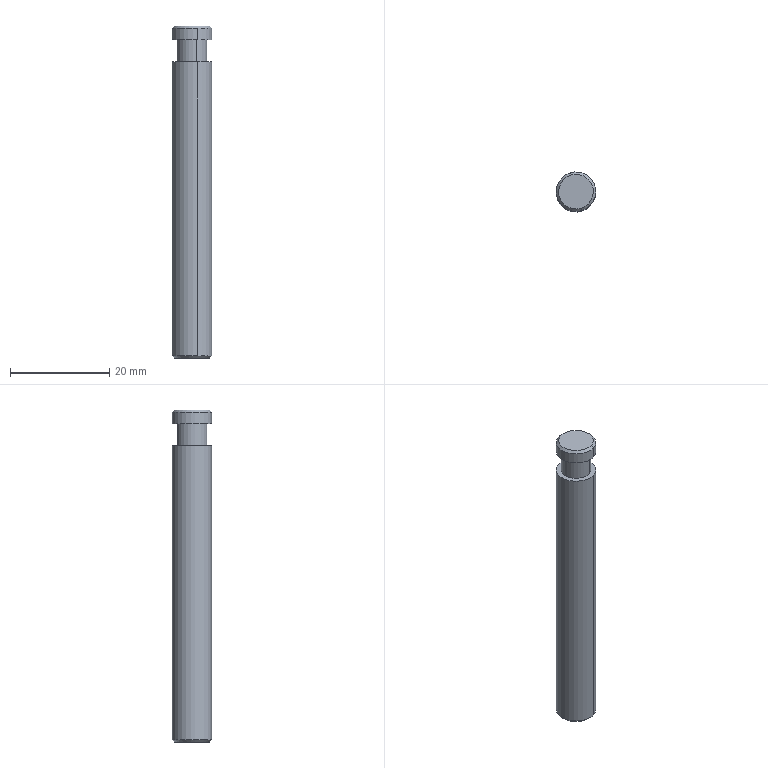Component | SolidWorks | 170423A4-ConveyorBeltIdlerAssembly1-1_170423A4-IdlerFixedAxis1-1 | 1 solid | 14 faces | box 8 x 8 x 67 mm | volume 3263 mm3 | cylinder 6 | cone 4 | plane 4 | commonest cylinder face diameters 8 x4 6 x2
build123d program:
from build123d import *

# Parameters (mm, degrees)
SKETCH1_R           = 4
BOSS_EXTRUDE1_DEPTH = 67
SKETCH2_W           = 4.5
SKETCH2_H           = 1
CHAMFER1_SIZE       = 0.5


with BuildPart() as part:
    # Sketch1 → Boss-Extrude1 (new body)
    with BuildSketch(Plane.XY):
        Circle(SKETCH1_R)
    extrude(amount=BOSS_EXTRUDE1_DEPTH)

    # Sketch2 → Cut-Revolve1 (revolve, cut)
    with BuildSketch(Plane(origin=(0, 0, 0), x_dir=(0, 0, -1), z_dir=(1, 0, 0)), mode=Mode.PRIVATE) as cut_revolve1_sk:
        with Locations((-62, 3.5)):
            Rectangle(SKETCH2_W, SKETCH2_H)
    revolve(cut_revolve1_sk.sketch.rotate(Axis((0, 0, 0), (0, 0, -1)), 90), axis=Axis((0, 0, 0), (0, 0, -1)), mode=Mode.SUBTRACT)

    # Chamfer1
    chamfer1_edges = [part.edges().sort_by_distance(p)[0] for p in [
        (-4, 0, 0),
        (-4, 0, 67),
    ]]
    chamfer(chamfer1_edges, length=CHAMFER1_SIZE)


solid = part.part

# Placed as in the assembly
solid = solid.moved(Location((14.754, -95.788, 415), (0, 0, 0)))
STEP:
#1=COLOUR_RGB('',0.7922,0.8196,0.9333);
#2=FILL_AREA_STYLE_COLOUR('',#1);
#3=FILL_AREA_STYLE('',(#2));
#4=SURFACE_STYLE_FILL_AREA(#3);
#5=SURFACE_SIDE_STYLE('',(#4));
#6=SURFACE_STYLE_USAGE(.BOTH.,#5);
#7=PRESENTATION_STYLE_ASSIGNMENT((#6));
#8=CARTESIAN_POINT('',(0.6212,-3.903,16.339));
#9=VERTEX_POINT('',#8);
#10=CARTESIAN_POINT('',(0.5405,-3.639,16.339));
#11=VERTEX_POINT('',#10);
#12=CARTESIAN_POINT('',(0.5808,-3.771,16.339));
#13=DIRECTION('',(0.,0.,-1.));
#14=DIRECTION('',(-0.293,0.9561,0.));
#15=AXIS2_PLACEMENT_3D('',#12,#13,#14);
#16=CIRCLE('',#15,0.1378);
#17=EDGE_CURVE('',#9,#11,#16,.T.);
#18=ORIENTED_EDGE('',*,*,#17,.F.);
#19=CARTESIAN_POINT('',(0.627,-3.922,16.358));
#20=VERTEX_POINT('',#19);
#21=CARTESIAN_POINT('',(0.627,-3.922,16.358));
#22=DIRECTION('',(0.2072,-0.6761,0.7071));
#23=VECTOR('',#22,39.37);
#24=LINE('',#21,#23);
#25=EDGE_CURVE('',#9,#20,#24,.T.);
#26=ORIENTED_EDGE('',*,*,#25,.T.);
#27=CARTESIAN_POINT('',(0.5347,-3.621,16.358));
#28=VERTEX_POINT('',#27);
#29=CARTESIAN_POINT('',(0.5808,-3.771,16.358));
#30=DIRECTION('',(0.,0.,1.));
#31=DIRECTION('',(-0.293,0.9561,0.));
#32=AXIS2_PLACEMENT_3D('',#29,#30,#31);
#33=CIRCLE('',#32,0.1575);
#34=EDGE_CURVE('',#28,#20,#33,.T.);
#35=ORIENTED_EDGE('',*,*,#34,.F.);
#36=CARTESIAN_POINT('',(0.5347,-3.621,16.358));
#37=DIRECTION('',(-0.2072,0.6761,0.7071));
#38=VECTOR('',#37,39.37);
#39=LINE('',#36,#38);
#40=EDGE_CURVE('',#11,#28,#39,.T.);
#41=ORIENTED_EDGE('',*,*,#40,.F.);
#42=EDGE_LOOP('',(#18,#26,#35,#41));
#43=FACE_OUTER_BOUND('',#42,.T.);
#44=CARTESIAN_POINT('',(0.5808,-3.771,16.358));
#45=DIRECTION('',(0.,0.,1.));
#46=DIRECTION('',(-0.293,0.9561,0.));
#47=AXIS2_PLACEMENT_3D('',#44,#45,#46);
#48=CONICAL_SURFACE('',#47,0.1575,0.7854);
#49=ADVANCED_FACE('',(#43),#48,.T.);
#50=CARTESIAN_POINT('',(0.5405,-3.639,18.976));
#51=VERTEX_POINT('',#50);
#52=CARTESIAN_POINT('',(0.6212,-3.903,18.976));
#53=VERTEX_POINT('',#52);
#54=CARTESIAN_POINT('',(0.5808,-3.771,18.976));
#55=DIRECTION('',(0.,0.,1.));
#56=DIRECTION('',(-0.293,0.9561,0.));
#57=AXIS2_PLACEMENT_3D('',#54,#55,#56);
#58=CIRCLE('',#57,0.1378);
#59=EDGE_CURVE('',#51,#53,#58,.T.);
#60=ORIENTED_EDGE('',*,*,#59,.F.);
#61=CARTESIAN_POINT('',(0.5347,-3.621,18.957));
#62=VERTEX_POINT('',#61);
#63=CARTESIAN_POINT('',(0.5405,-3.639,18.976));
#64=DIRECTION('',(-0.2072,0.6761,-0.7071));
#65=VECTOR('',#64,39.37);
#66=LINE('',#63,#65);
#67=EDGE_CURVE('',#51,#62,#66,.T.);
#68=ORIENTED_EDGE('',*,*,#67,.T.);
#69=CARTESIAN_POINT('',(0.627,-3.922,18.957));
#70=VERTEX_POINT('',#69);
#71=CARTESIAN_POINT('',(0.5808,-3.771,18.957));
#72=DIRECTION('',(0.,0.,-1.));
#73=DIRECTION('',(-0.293,0.9561,0.));
#74=AXIS2_PLACEMENT_3D('',#71,#72,#73);
#75=CIRCLE('',#74,0.1575);
#76=EDGE_CURVE('',#70,#62,#75,.T.);
#77=ORIENTED_EDGE('',*,*,#76,.F.);
#78=CARTESIAN_POINT('',(0.6212,-3.903,18.976));
#79=DIRECTION('',(0.2072,-0.6761,-0.7071));
#80=VECTOR('',#79,39.37);
#81=LINE('',#78,#80);
#82=EDGE_CURVE('',#53,#70,#81,.T.);
#83=ORIENTED_EDGE('',*,*,#82,.F.);
#84=EDGE_LOOP('',(#60,#68,#77,#83));
#85=FACE_OUTER_BOUND('',#84,.T.);
#86=CARTESIAN_POINT('',(0.5808,-3.771,18.976));
#87=DIRECTION('',(0.,0.,-1.));
#88=DIRECTION('',(0.293,-0.9561,0.));
#89=AXIS2_PLACEMENT_3D('',#86,#87,#88);
#90=CONICAL_SURFACE('',#89,0.1378,0.7854);
#91=ADVANCED_FACE('',(#85),#90,.T.);
#92=CARTESIAN_POINT('',(0.5347,-3.621,18.691));
#93=VERTEX_POINT('',#92);
#94=CARTESIAN_POINT('',(0.627,-3.922,18.691));
#95=VERTEX_POINT('',#94);
#96=CARTESIAN_POINT('',(0.5808,-3.771,18.691));
#97=DIRECTION('',(0.,0.,1.));
#98=DIRECTION('',(-0.293,0.9561,0.));
#99=AXIS2_PLACEMENT_3D('',#96,#97,#98);
#100=CIRCLE('',#99,0.1575);
#101=EDGE_CURVE('',#93,#95,#100,.T.);
#102=ORIENTED_EDGE('',*,*,#101,.F.);
#103=CARTESIAN_POINT('',(0.5347,-3.621,18.976));
#104=DIRECTION('',(0.,0.,-1.));
#105=VECTOR('',#104,39.37);
#106=LINE('',#103,#105);
#107=EDGE_CURVE('',#93,#28,#106,.T.);
#108=ORIENTED_EDGE('',*,*,#107,.T.);
#109=ORIENTED_EDGE('',*,*,#34,.T.);
#110=CARTESIAN_POINT('',(0.627,-3.922,18.976));
#111=DIRECTION('',(0.,0.,-1.));
#112=VECTOR('',#111,39.37);
#113=LINE('',#110,#112);
#114=EDGE_CURVE('',#95,#20,#113,.T.);
#115=ORIENTED_EDGE('',*,*,#114,.F.);
#116=EDGE_LOOP('',(#102,#108,#109,#115));
#117=FACE_OUTER_BOUND('',#116,.T.);
#118=CARTESIAN_POINT('',(0.5808,-3.771,18.976));
#119=DIRECTION('',(0.,0.,-1.));
#120=DIRECTION('',(0.293,-0.9561,0.));
#121=AXIS2_PLACEMENT_3D('',#118,#119,#120);
#122=CYLINDRICAL_SURFACE('',#121,0.1575);
#123=ADVANCED_FACE('',(#117),#122,.T.);
#124=CARTESIAN_POINT('',(0.5462,-3.658,18.691));
#125=VERTEX_POINT('',#124);
#126=CARTESIAN_POINT('',(0.6155,-3.884,18.691));
#127=VERTEX_POINT('',#126);
#128=CARTESIAN_POINT('',(0.5808,-3.771,18.691));
#129=DIRECTION('',(0.,0.,1.));
#130=DIRECTION('',(-0.293,0.9561,0.));
#131=AXIS2_PLACEMENT_3D('',#128,#129,#130);
#132=CIRCLE('',#131,0.1181);
#133=EDGE_CURVE('',#125,#127,#132,.T.);
#134=ORIENTED_EDGE('',*,*,#133,.T.);
#135=CARTESIAN_POINT('',(0.6155,-3.884,18.868));
#136=VERTEX_POINT('',#135);
#137=CARTESIAN_POINT('',(0.6155,-3.884,16.339));
#138=DIRECTION('',(0.,0.,1.));
#139=VECTOR('',#138,39.37);
#140=LINE('',#137,#139);
#141=EDGE_CURVE('',#127,#136,#140,.T.);
#142=ORIENTED_EDGE('',*,*,#141,.T.);
#143=CARTESIAN_POINT('',(0.5462,-3.658,18.868));
#144=VERTEX_POINT('',#143);
#145=CARTESIAN_POINT('',(0.5808,-3.771,18.868));
#146=DIRECTION('',(0.,0.,1.));
#147=DIRECTION('',(-0.293,0.9561,0.));
#148=AXIS2_PLACEMENT_3D('',#145,#146,#147);
#149=CIRCLE('',#148,0.1181);
#150=EDGE_CURVE('',#144,#136,#149,.T.);
#151=ORIENTED_EDGE('',*,*,#150,.F.);
#152=CARTESIAN_POINT('',(0.5462,-3.658,16.339));
#153=DIRECTION('',(0.,0.,1.));
#154=VECTOR('',#153,39.37);
#155=LINE('',#152,#154);
#156=EDGE_CURVE('',#125,#144,#155,.T.);
#157=ORIENTED_EDGE('',*,*,#156,.F.);
#158=EDGE_LOOP('',(#134,#142,#151,#157));
#159=FACE_OUTER_BOUND('',#158,.T.);
#160=CARTESIAN_POINT('',(0.5808,-3.771,16.339));
#161=DIRECTION('',(0.,0.,1.));
#162=DIRECTION('',(-0.293,0.9561,0.));
#163=AXIS2_PLACEMENT_3D('',#160,#161,#162);
#164=CYLINDRICAL_SURFACE('',#163,0.1181);
#165=ADVANCED_FACE('',(#159),#164,.T.);
#166=ORIENTED_EDGE('',*,*,#76,.T.);
#167=CARTESIAN_POINT('',(0.5347,-3.621,18.868));
#168=VERTEX_POINT('',#167);
#169=CARTESIAN_POINT('',(0.5347,-3.621,18.976));
#170=DIRECTION('',(0.,0.,-1.));
#171=VECTOR('',#170,39.37);
#172=LINE('',#169,#171);
#173=EDGE_CURVE('',#62,#168,#172,.T.);
#174=ORIENTED_EDGE('',*,*,#173,.T.);
#175=CARTESIAN_POINT('',(0.627,-3.922,18.868));
#176=VERTEX_POINT('',#175);
#177=CARTESIAN_POINT('',(0.5808,-3.771,18.868));
#178=DIRECTION('',(0.,0.,1.));
#179=DIRECTION('',(-0.293,0.9561,0.));
#180=AXIS2_PLACEMENT_3D('',#177,#178,#179);
#181=CIRCLE('',#180,0.1575);
#182=EDGE_CURVE('',#168,#176,#181,.T.);
#183=ORIENTED_EDGE('',*,*,#182,.T.);
#184=CARTESIAN_POINT('',(0.627,-3.922,18.976));
#185=DIRECTION('',(0.,0.,-1.));
#186=VECTOR('',#185,39.37);
#187=LINE('',#184,#186);
#188=EDGE_CURVE('',#70,#176,#187,.T.);
#189=ORIENTED_EDGE('',*,*,#188,.F.);
#190=EDGE_LOOP('',(#166,#174,#183,#189));
#191=FACE_OUTER_BOUND('',#190,.T.);
#192=CARTESIAN_POINT('',(0.5808,-3.771,18.976));
#193=DIRECTION('',(0.,0.,-1.));
#194=DIRECTION('',(0.293,-0.9561,0.));
#195=AXIS2_PLACEMENT_3D('',#192,#193,#194);
#196=CYLINDRICAL_SURFACE('',#195,0.1575);
#197=ADVANCED_FACE('',(#191),#196,.T.);
#198=ORIENTED_EDGE('',*,*,#173,.F.);
#199=CARTESIAN_POINT('',(0.5808,-3.771,18.957));
#200=DIRECTION('',(0.,0.,-1.));
#201=DIRECTION('',(-0.293,0.9561,0.));
#202=AXIS2_PLACEMENT_3D('',#199,#200,#201);
#203=CIRCLE('',#202,0.1575);
#204=EDGE_CURVE('',#62,#70,#203,.T.);
#205=ORIENTED_EDGE('',*,*,#204,.T.);
#206=ORIENTED_EDGE('',*,*,#188,.T.);
#207=CARTESIAN_POINT('',(0.5808,-3.771,18.868));
#208=DIRECTION('',(0.,0.,1.));
#209=DIRECTION('',(-0.293,0.9561,0.));
#210=AXIS2_PLACEMENT_3D('',#207,#208,#209);
#211=CIRCLE('',#210,0.1575);
#212=EDGE_CURVE('',#176,#168,#211,.T.);
#213=ORIENTED_EDGE('',*,*,#212,.T.);
#214=EDGE_LOOP('',(#198,#205,#206,#213));
#215=FACE_OUTER_BOUND('',#214,.T.);
#216=CARTESIAN_POINT('',(0.5808,-3.771,18.976));
#217=DIRECTION('',(0.,0.,-1.));
#218=DIRECTION('',(0.293,-0.9561,0.));
#219=AXIS2_PLACEMENT_3D('',#216,#217,#218);
#220=CYLINDRICAL_SURFACE('',#219,0.1575);
#221=ADVANCED_FACE('',(#215),#220,.T.);
#222=CARTESIAN_POINT('',(0.5808,-3.771,18.976));
#223=DIRECTION('',(0.,0.,1.));
#224=DIRECTION('',(-0.293,0.9561,0.));
#225=AXIS2_PLACEMENT_3D('',#222,#223,#224);
#226=CIRCLE('',#225,0.1378);
#227=EDGE_CURVE('',#53,#51,#226,.T.);
#228=ORIENTED_EDGE('',*,*,#227,.T.);
#229=ORIENTED_EDGE('',*,*,#59,.T.);
#230=EDGE_LOOP('',(#228,#229));
#231=FACE_OUTER_BOUND('',#230,.T.);
#232=CARTESIAN_POINT('',(0.5808,-3.771,18.976));
#233=DIRECTION('',(0.,0.,1.));
#234=DIRECTION('',(-0.293,0.9561,0.));
#235=AXIS2_PLACEMENT_3D('',#232,#233,#234);
#236=PLANE('',#235);
#237=ADVANCED_FACE('',(#231),#236,.T.);
#238=ORIENTED_EDGE('',*,*,#150,.T.);
#239=CARTESIAN_POINT('',(0.5808,-3.771,18.868));
#240=DIRECTION('',(0.,0.,1.));
#241=DIRECTION('',(-0.293,0.9561,0.));
#242=AXIS2_PLACEMENT_3D('',#239,#240,#241);
#243=CIRCLE('',#242,0.1181);
#244=EDGE_CURVE('',#136,#144,#243,.T.);
#245=ORIENTED_EDGE('',*,*,#244,.T.);
#246=EDGE_LOOP('',(#238,#245));
#247=FACE_BOUND('',#246,.T.);
#248=ORIENTED_EDGE('',*,*,#212,.F.);
#249=ORIENTED_EDGE('',*,*,#182,.F.);
#250=EDGE_LOOP('',(#248,#249));
#251=FACE_OUTER_BOUND('',#250,.T.);
#252=CARTESIAN_POINT('',(0.4303,-3.817,18.868));
#253=DIRECTION('',(0.,0.,-1.));
#254=DIRECTION('',(0.293,-0.9561,0.));
#255=AXIS2_PLACEMENT_3D('',#252,#253,#254);
#256=PLANE('',#255);
#257=ADVANCED_FACE('',(#247,#251),#256,.T.);
#258=ORIENTED_EDGE('',*,*,#141,.F.);
#259=CARTESIAN_POINT('',(0.5808,-3.771,18.691));
#260=DIRECTION('',(0.,0.,1.));
#261=DIRECTION('',(-0.293,0.9561,0.));
#262=AXIS2_PLACEMENT_3D('',#259,#260,#261);
#263=CIRCLE('',#262,0.1181);
#264=EDGE_CURVE('',#127,#125,#263,.T.);
#265=ORIENTED_EDGE('',*,*,#264,.T.);
#266=ORIENTED_EDGE('',*,*,#156,.T.);
#267=ORIENTED_EDGE('',*,*,#244,.F.);
#268=EDGE_LOOP('',(#258,#265,#266,#267));
#269=FACE_OUTER_BOUND('',#268,.T.);
#270=CARTESIAN_POINT('',(0.5808,-3.771,16.339));
#271=DIRECTION('',(0.,0.,1.));
#272=DIRECTION('',(-0.293,0.9561,0.));
#273=AXIS2_PLACEMENT_3D('',#270,#271,#272);
#274=CYLINDRICAL_SURFACE('',#273,0.1181);
#275=ADVANCED_FACE('',(#269),#274,.T.);
#276=CARTESIAN_POINT('',(0.5808,-3.771,18.691));
#277=DIRECTION('',(0.,0.,1.));
#278=DIRECTION('',(-0.293,0.9561,0.));
#279=AXIS2_PLACEMENT_3D('',#276,#277,#278);
#280=CIRCLE('',#279,0.1575);
#281=EDGE_CURVE('',#95,#93,#280,.T.);
#282=ORIENTED_EDGE('',*,*,#281,.T.);
#283=ORIENTED_EDGE('',*,*,#101,.T.);
#284=EDGE_LOOP('',(#282,#283));
#285=FACE_OUTER_BOUND('',#284,.T.);
#286=ORIENTED_EDGE('',*,*,#133,.F.);
#287=ORIENTED_EDGE('',*,*,#264,.F.);
#288=EDGE_LOOP('',(#286,#287));
#289=FACE_BOUND('',#288,.T.);
#290=CARTESIAN_POINT('',(0.4303,-3.817,18.691));
#291=DIRECTION('',(0.,0.,1.));
#292=DIRECTION('',(-0.293,0.9561,0.));
#293=AXIS2_PLACEMENT_3D('',#290,#291,#292);
#294=PLANE('',#293);
#295=ADVANCED_FACE('',(#285,#289),#294,.T.);
#296=CARTESIAN_POINT('',(0.5808,-3.771,16.339));
#297=DIRECTION('',(0.,0.,-1.));
#298=DIRECTION('',(-0.293,0.9561,0.));
#299=AXIS2_PLACEMENT_3D('',#296,#297,#298);
#300=CIRCLE('',#299,0.1378);
#301=EDGE_CURVE('',#11,#9,#300,.T.);
#302=ORIENTED_EDGE('',*,*,#301,.T.);
#303=ORIENTED_EDGE('',*,*,#17,.T.);
#304=EDGE_LOOP('',(#302,#303));
#305=FACE_OUTER_BOUND('',#304,.T.);
#306=CARTESIAN_POINT('',(0.5808,-3.771,16.339));
#307=DIRECTION('',(0.,0.,1.));
#308=DIRECTION('',(-0.293,0.9561,0.));
#309=AXIS2_PLACEMENT_3D('',#306,#307,#308);
#310=PLANE('',#309);
#311=ADVANCED_FACE('',(#305),#310,.F.);
#312=ORIENTED_EDGE('',*,*,#107,.F.);
#313=ORIENTED_EDGE('',*,*,#281,.F.);
#314=ORIENTED_EDGE('',*,*,#114,.T.);
#315=CARTESIAN_POINT('',(0.5808,-3.771,16.358));
#316=DIRECTION('',(0.,0.,1.));
#317=DIRECTION('',(-0.293,0.9561,0.));
#318=AXIS2_PLACEMENT_3D('',#315,#316,#317);
#319=CIRCLE('',#318,0.1575);
#320=EDGE_CURVE('',#20,#28,#319,.T.);
#321=ORIENTED_EDGE('',*,*,#320,.T.);
#322=EDGE_LOOP('',(#312,#313,#314,#321));
#323=FACE_OUTER_BOUND('',#322,.T.);
#324=CARTESIAN_POINT('',(0.5808,-3.771,18.976));
#325=DIRECTION('',(0.,0.,-1.));
#326=DIRECTION('',(0.293,-0.9561,0.));
#327=AXIS2_PLACEMENT_3D('',#324,#325,#326);
#328=CYLINDRICAL_SURFACE('',#327,0.1575);
#329=ADVANCED_FACE('',(#323),#328,.T.);
#330=ORIENTED_EDGE('',*,*,#67,.F.);
#331=ORIENTED_EDGE('',*,*,#227,.F.);
#332=ORIENTED_EDGE('',*,*,#82,.T.);
#333=ORIENTED_EDGE('',*,*,#204,.F.);
#334=EDGE_LOOP('',(#330,#331,#332,#333));
#335=FACE_OUTER_BOUND('',#334,.T.);
#336=CARTESIAN_POINT('',(0.5808,-3.771,18.976));
#337=DIRECTION('',(0.,0.,-1.));
#338=DIRECTION('',(0.293,-0.9561,0.));
#339=AXIS2_PLACEMENT_3D('',#336,#337,#338);
#340=CONICAL_SURFACE('',#339,0.1378,0.7854);
#341=ADVANCED_FACE('',(#335),#340,.T.);
#342=ORIENTED_EDGE('',*,*,#25,.F.);
#343=ORIENTED_EDGE('',*,*,#301,.F.);
#344=ORIENTED_EDGE('',*,*,#40,.T.);
#345=ORIENTED_EDGE('',*,*,#320,.F.);
#346=EDGE_LOOP('',(#342,#343,#344,#345));
#347=FACE_OUTER_BOUND('',#346,.T.);
#348=CARTESIAN_POINT('',(0.5808,-3.771,16.358));
#349=DIRECTION('',(0.,0.,1.));
#350=DIRECTION('',(-0.293,0.9561,0.));
#351=AXIS2_PLACEMENT_3D('',#348,#349,#350);
#352=CONICAL_SURFACE('',#351,0.1575,0.7854);
#353=ADVANCED_FACE('',(#347),#352,.T.);
#354=CLOSED_SHELL('',(#49,#91,#123,#165,#197,#221,#237,#257,#275,#295,#311,#329,#341,#353));
#355=MANIFOLD_SOLID_BREP('',#354);
#356=STYLED_ITEM('',(#7),#355);
#357=PRESENTATION_LAYER_ASSIGNMENT('','',(#356));
#358=(LENGTH_UNIT()NAMED_UNIT(*)SI_UNIT($,.METRE.));
#359=LENGTH_MEASURE_WITH_UNIT(LENGTH_MEASURE(0.0254),#358);
#360=DIMENSIONAL_EXPONENTS(1.,0.,0.,0.,0.,0.,0.);
#361=(CONVERSION_BASED_UNIT('',#359)LENGTH_UNIT()NAMED_UNIT(#360));
#362=UNCERTAINTY_MEASURE_WITH_UNIT(LENGTH_MEASURE(0.00001),#361,'','');
#363=(NAMED_UNIT(*)PLANE_ANGLE_UNIT()SI_UNIT($,.RADIAN.));
#364=(NAMED_UNIT(*)SI_UNIT($,.STERADIAN.)SOLID_ANGLE_UNIT());
#365=(GEOMETRIC_REPRESENTATION_CONTEXT(3)GLOBAL_UNCERTAINTY_ASSIGNED_CONTEXT((#362))GLOBAL_UNIT_ASSIGNED_CONTEXT((#361,#363,#364))REPRESENTATION_CONTEXT('',''));
#366=MECHANICAL_DESIGN_GEOMETRIC_PRESENTATION_REPRESENTATION('',(#356),#365);
#367=CARTESIAN_POINT('',(0.,0.,0.));
#368=DIRECTION('',(0.,0.,1.));
#369=DIRECTION('',(1.,0.,0.));
#370=AXIS2_PLACEMENT_3D('',#367,#368,#369);
#371=(LENGTH_UNIT()NAMED_UNIT(*)SI_UNIT($,.METRE.));
#372=LENGTH_MEASURE_WITH_UNIT(LENGTH_MEASURE(0.0254),#371);
#373=DIMENSIONAL_EXPONENTS(1.,0.,0.,0.,0.,0.,0.);
#374=(CONVERSION_BASED_UNIT('',#372)LENGTH_UNIT()NAMED_UNIT(#373));
#375=UNCERTAINTY_MEASURE_WITH_UNIT(LENGTH_MEASURE(0.00001),#374,'','');
#376=(NAMED_UNIT(*)PLANE_ANGLE_UNIT()SI_UNIT($,.RADIAN.));
#377=(NAMED_UNIT(*)SI_UNIT($,.STERADIAN.)SOLID_ANGLE_UNIT());
#378=(GEOMETRIC_REPRESENTATION_CONTEXT(3)GLOBAL_UNCERTAINTY_ASSIGNED_CONTEXT((#375))GLOBAL_UNIT_ASSIGNED_CONTEXT((#374,#376,#377))REPRESENTATION_CONTEXT('',''));
#379=ADVANCED_BREP_SHAPE_REPRESENTATION('',(#355,#370),#378);